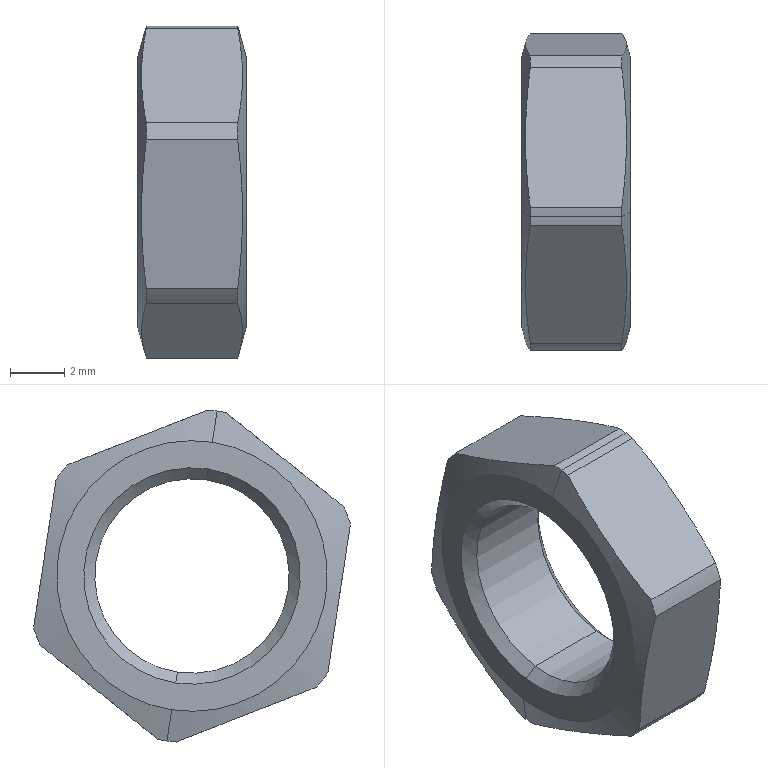Component | SolidWorks | CCDJSACA0806-1-2_CCDJSACA-0806-1_NT-3 | 1 solid | 25 faces | box 4 x 11.71 x 12.27 mm | volume 245 mm3 | cylinder 9 | cone 8 | plane 8 | commonest cylinder face diameters 12.325 x7 7.188 x2
STEP:
#1=CARTESIAN_POINT('',(-8.728,15.708,-2.258));
#2=VERTEX_POINT('',#1);
#3=CARTESIAN_POINT('',(-8.728,15.694,-2.26));
#4=VERTEX_POINT('',#3);
#5=CARTESIAN_POINT('',(-8.728,15.731,-2.5));
#6=DIRECTION('',(1.,-0.,-0.));
#7=DIRECTION('',(0.,-0.1502,0.9887));
#8=AXIS2_PLACEMENT_3D('',#5,#6,#7);
#9=CIRCLE('',#8,0.2426);
#10=EDGE_CURVE('',#2,#4,#9,.T.);
#11=ORIENTED_EDGE('',*,*,#10,.T.);
#12=CARTESIAN_POINT('',(-8.595,15.694,-2.26));
#13=VERTEX_POINT('',#12);
#14=CARTESIAN_POINT('',(-8.898,15.694,-2.26));
#15=DIRECTION('',(1.,-0.,-0.));
#16=VECTOR('',#15,39.37);
#17=LINE('',#14,#16);
#18=EDGE_CURVE('',#4,#13,#17,.T.);
#19=ORIENTED_EDGE('',*,*,#18,.T.);
#20=CARTESIAN_POINT('',(-8.595,15.708,-2.258));
#21=VERTEX_POINT('',#20);
#22=CARTESIAN_POINT('',(-8.595,15.731,-2.5));
#23=DIRECTION('',(-1.,0.,0.));
#24=DIRECTION('',(0.,0.1502,-0.9887));
#25=AXIS2_PLACEMENT_3D('',#22,#23,#24);
#26=CIRCLE('',#25,0.2426);
#27=EDGE_CURVE('',#13,#21,#26,.T.);
#28=ORIENTED_EDGE('',*,*,#27,.T.);
#29=CARTESIAN_POINT('',(-8.898,15.708,-2.258));
#30=DIRECTION('',(1.,-0.,-0.));
#31=VECTOR('',#30,39.37);
#32=LINE('',#29,#31);
#33=EDGE_CURVE('',#2,#21,#32,.T.);
#34=ORIENTED_EDGE('',*,*,#33,.F.);
#35=EDGE_LOOP('',(#11,#19,#28,#34));
#36=FACE_OUTER_BOUND('',#35,.T.);
#37=CARTESIAN_POINT('',(-8.898,15.731,-2.5));
#38=DIRECTION('',(1.,-0.,-0.));
#39=DIRECTION('',(0.,-0.1502,0.9887));
#40=AXIS2_PLACEMENT_3D('',#37,#38,#39);
#41=CYLINDRICAL_SURFACE('',#40,0.2426);
#42=ADVANCED_FACE('',(#36),#41,.T.);
#43=CARTESIAN_POINT('',(-8.724,15.752,-2.64));
#44=VERTEX_POINT('',#43);
#45=CARTESIAN_POINT('',(-8.724,15.71,-2.36));
#46=VERTEX_POINT('',#45);
#47=CARTESIAN_POINT('',(-8.724,15.731,-2.5));
#48=DIRECTION('',(1.,-0.,-0.));
#49=DIRECTION('',(0.,-0.1502,0.9887));
#50=AXIS2_PLACEMENT_3D('',#47,#48,#49);
#51=CIRCLE('',#50,0.1415);
#52=EDGE_CURVE('',#44,#46,#51,.T.);
#53=ORIENTED_EDGE('',*,*,#52,.T.);
#54=CARTESIAN_POINT('',(-8.74,15.707,-2.344));
#55=VERTEX_POINT('',#54);
#56=CARTESIAN_POINT('',(-8.724,15.71,-2.36));
#57=DIRECTION('',(-0.7071,-0.1062,0.6991));
#58=VECTOR('',#57,39.37);
#59=LINE('',#56,#58);
#60=EDGE_CURVE('',#46,#55,#59,.T.);
#61=ORIENTED_EDGE('',*,*,#60,.T.);
#62=CARTESIAN_POINT('',(-8.74,15.755,-2.656));
#63=VERTEX_POINT('',#62);
#64=CARTESIAN_POINT('',(-8.74,15.731,-2.5));
#65=DIRECTION('',(1.,-0.,-0.));
#66=DIRECTION('',(0.,-0.1502,0.9887));
#67=AXIS2_PLACEMENT_3D('',#64,#65,#66);
#68=CIRCLE('',#67,0.1575);
#69=EDGE_CURVE('',#63,#55,#68,.T.);
#70=ORIENTED_EDGE('',*,*,#69,.F.);
#71=CARTESIAN_POINT('',(-8.724,15.752,-2.64));
#72=DIRECTION('',(-0.7071,0.1062,-0.6991));
#73=VECTOR('',#72,39.37);
#74=LINE('',#71,#73);
#75=EDGE_CURVE('',#44,#63,#74,.T.);
#76=ORIENTED_EDGE('',*,*,#75,.F.);
#77=EDGE_LOOP('',(#53,#61,#70,#76));
#78=FACE_OUTER_BOUND('',#77,.T.);
#79=CARTESIAN_POINT('',(-8.724,15.731,-2.5));
#80=DIRECTION('',(-1.,0.,0.));
#81=DIRECTION('',(0.,0.1502,-0.9887));
#82=AXIS2_PLACEMENT_3D('',#79,#80,#81);
#83=CONICAL_SURFACE('',#82,0.1415,0.7854);
#84=ADVANCED_FACE('',(#78),#83,.F.);
#85=ORIENTED_EDGE('',*,*,#52,.F.);
#86=CARTESIAN_POINT('',(-8.599,15.752,-2.64));
#87=VERTEX_POINT('',#86);
#88=CARTESIAN_POINT('',(-8.74,15.752,-2.64));
#89=DIRECTION('',(1.,-0.,-0.));
#90=VECTOR('',#89,39.37);
#91=LINE('',#88,#90);
#92=EDGE_CURVE('',#44,#87,#91,.T.);
#93=ORIENTED_EDGE('',*,*,#92,.T.);
#94=CARTESIAN_POINT('',(-8.599,15.71,-2.36));
#95=VERTEX_POINT('',#94);
#96=CARTESIAN_POINT('',(-8.599,15.731,-2.5));
#97=DIRECTION('',(1.,-0.,-0.));
#98=DIRECTION('',(0.,-0.1502,0.9887));
#99=AXIS2_PLACEMENT_3D('',#96,#97,#98);
#100=CIRCLE('',#99,0.1415);
#101=EDGE_CURVE('',#87,#95,#100,.T.);
#102=ORIENTED_EDGE('',*,*,#101,.T.);
#103=CARTESIAN_POINT('',(-8.74,15.71,-2.36));
#104=DIRECTION('',(1.,-0.,-0.));
#105=VECTOR('',#104,39.37);
#106=LINE('',#103,#105);
#107=EDGE_CURVE('',#46,#95,#106,.T.);
#108=ORIENTED_EDGE('',*,*,#107,.F.);
#109=EDGE_LOOP('',(#85,#93,#102,#108));
#110=FACE_OUTER_BOUND('',#109,.T.);
#111=CARTESIAN_POINT('',(-8.74,15.731,-2.5));
#112=DIRECTION('',(1.,-0.,-0.));
#113=DIRECTION('',(0.,-0.1502,0.9887));
#114=AXIS2_PLACEMENT_3D('',#111,#112,#113);
#115=CYLINDRICAL_SURFACE('',#114,0.1415);
#116=ADVANCED_FACE('',(#110),#115,.F.);
#117=ORIENTED_EDGE('',*,*,#101,.F.);
#118=CARTESIAN_POINT('',(-8.583,15.755,-2.656));
#119=VERTEX_POINT('',#118);
#120=CARTESIAN_POINT('',(-8.583,15.755,-2.656));
#121=DIRECTION('',(0.7071,0.1062,-0.6991));
#122=VECTOR('',#121,39.37);
#123=LINE('',#120,#122);
#124=EDGE_CURVE('',#87,#119,#123,.T.);
#125=ORIENTED_EDGE('',*,*,#124,.T.);
#126=CARTESIAN_POINT('',(-8.583,15.707,-2.344));
#127=VERTEX_POINT('',#126);
#128=CARTESIAN_POINT('',(-8.583,15.731,-2.5));
#129=DIRECTION('',(1.,-0.,-0.));
#130=DIRECTION('',(0.,-0.1502,0.9887));
#131=AXIS2_PLACEMENT_3D('',#128,#129,#130);
#132=CIRCLE('',#131,0.1575);
#133=EDGE_CURVE('',#119,#127,#132,.T.);
#134=ORIENTED_EDGE('',*,*,#133,.T.);
#135=CARTESIAN_POINT('',(-8.583,15.707,-2.344));
#136=DIRECTION('',(0.7071,-0.1062,0.6991));
#137=VECTOR('',#136,39.37);
#138=LINE('',#135,#137);
#139=EDGE_CURVE('',#95,#127,#138,.T.);
#140=ORIENTED_EDGE('',*,*,#139,.F.);
#141=EDGE_LOOP('',(#117,#125,#134,#140));
#142=FACE_OUTER_BOUND('',#141,.T.);
#143=CARTESIAN_POINT('',(-8.583,15.731,-2.5));
#144=DIRECTION('',(1.,-0.,-0.));
#145=DIRECTION('',(0.,-0.1502,0.9887));
#146=AXIS2_PLACEMENT_3D('',#143,#144,#145);
#147=CONICAL_SURFACE('',#146,0.1575,0.7854);
#148=ADVANCED_FACE('',(#142),#147,.F.);
#149=CARTESIAN_POINT('',(-8.583,15.701,-2.305));
#150=VERTEX_POINT('',#149);
#151=CARTESIAN_POINT('',(-8.583,15.76,-2.695));
#152=VERTEX_POINT('',#151);
#153=CARTESIAN_POINT('',(-8.583,15.731,-2.5));
#154=DIRECTION('',(1.,-0.,-0.));
#155=DIRECTION('',(0.,-0.1502,0.9887));
#156=AXIS2_PLACEMENT_3D('',#153,#154,#155);
#157=CIRCLE('',#156,0.1969);
#158=EDGE_CURVE('',#150,#152,#157,.T.);
#159=ORIENTED_EDGE('',*,*,#158,.F.);
#160=CARTESIAN_POINT('',(-8.661,15.657,-2.015));
#161=DIRECTION('',(-0.2588,-0.1451,0.955));
#162=VECTOR('',#161,39.37);
#163=LINE('',#160,#162);
#164=EDGE_CURVE('',#150,#13,#163,.T.);
#165=ORIENTED_EDGE('',*,*,#164,.T.);
#166=CARTESIAN_POINT('',(-8.595,15.681,-2.263));
#167=VERTEX_POINT('',#166);
#168=CARTESIAN_POINT('',(-8.595,15.731,-2.5));
#169=DIRECTION('',(-1.,0.,0.));
#170=DIRECTION('',(0.,0.1502,-0.9887));
#171=AXIS2_PLACEMENT_3D('',#168,#169,#170);
#172=CIRCLE('',#171,0.2426);
#173=EDGE_CURVE('',#167,#13,#172,.T.);
#174=ORIENTED_EDGE('',*,*,#173,.F.);
#175=CARTESIAN_POINT('',(-8.595,15.51,-2.399));
#176=VERTEX_POINT('',#175);
#177=CARTESIAN_POINT('',(-8.595,15.51,-2.399));
#178=CARTESIAN_POINT('',(-8.591,15.539,-2.376));
#179=CARTESIAN_POINT('',(-8.585,15.596,-2.331));
#180=CARTESIAN_POINT('',(-8.591,15.653,-2.285));
#181=CARTESIAN_POINT('',(-8.595,15.681,-2.263));
#182=B_SPLINE_CURVE_WITH_KNOTS('',3,(#177,#178,#179,#180,#181),.UNSPECIFIED.,.F.,.F.,(4,1,4),(0.0003961,0.003176,0.005955),.UNSPECIFIED.);
#183=EDGE_CURVE('',#176,#167,#182,.T.);
#184=ORIENTED_EDGE('',*,*,#183,.F.);
#185=CARTESIAN_POINT('',(-8.595,15.5,-2.424));
#186=VERTEX_POINT('',#185);
#187=CARTESIAN_POINT('',(-8.595,15.731,-2.5));
#188=DIRECTION('',(-1.,0.,0.));
#189=DIRECTION('',(0.,0.1502,-0.9887));
#190=AXIS2_PLACEMENT_3D('',#187,#188,#189);
#191=CIRCLE('',#190,0.2426);
#192=EDGE_CURVE('',#186,#176,#191,.T.);
#193=ORIENTED_EDGE('',*,*,#192,.F.);
#194=CARTESIAN_POINT('',(-8.595,15.533,-2.641));
#195=VERTEX_POINT('',#194);
#196=CARTESIAN_POINT('',(-8.595,15.533,-2.641));
#197=CARTESIAN_POINT('',(-8.591,15.528,-2.605));
#198=CARTESIAN_POINT('',(-8.588,15.522,-2.568));
#199=CARTESIAN_POINT('',(-8.588,15.511,-2.496));
#200=CARTESIAN_POINT('',(-8.591,15.506,-2.46));
#201=CARTESIAN_POINT('',(-8.595,15.5,-2.424));
#202=B_SPLINE_CURVE_WITH_KNOTS('',3,(#196,#197,#198,#199,#200,#201),.UNSPECIFIED.,.F.,.F.,(4,2,4),(0.005822,0.00862,0.01142),.UNSPECIFIED.);
#203=EDGE_CURVE('',#195,#186,#202,.T.);
#204=ORIENTED_EDGE('',*,*,#203,.F.);
#205=CARTESIAN_POINT('',(-8.595,15.55,-2.662));
#206=VERTEX_POINT('',#205);
#207=CARTESIAN_POINT('',(-8.595,15.731,-2.5));
#208=DIRECTION('',(-1.,0.,0.));
#209=DIRECTION('',(0.,0.1502,-0.9887));
#210=AXIS2_PLACEMENT_3D('',#207,#208,#209);
#211=CIRCLE('',#210,0.2426);
#212=EDGE_CURVE('',#206,#195,#211,.T.);
#213=ORIENTED_EDGE('',*,*,#212,.F.);
#214=CARTESIAN_POINT('',(-8.595,15.754,-2.742));
#215=VERTEX_POINT('',#214);
#216=CARTESIAN_POINT('',(-8.595,15.754,-2.742));
#217=CARTESIAN_POINT('',(-8.591,15.72,-2.728));
#218=CARTESIAN_POINT('',(-8.585,15.652,-2.702));
#219=CARTESIAN_POINT('',(-8.591,15.584,-2.675));
#220=CARTESIAN_POINT('',(-8.595,15.55,-2.662));
#221=B_SPLINE_CURVE_WITH_KNOTS('',3,(#216,#217,#218,#219,#220),.UNSPECIFIED.,.F.,.F.,(4,1,4),(0.0003961,0.003176,0.005955),.UNSPECIFIED.);
#222=EDGE_CURVE('',#215,#206,#221,.T.);
#223=ORIENTED_EDGE('',*,*,#222,.F.);
#224=CARTESIAN_POINT('',(-8.595,15.767,-2.74));
#225=VERTEX_POINT('',#224);
#226=CARTESIAN_POINT('',(-8.595,15.731,-2.5));
#227=DIRECTION('',(-1.,0.,0.));
#228=DIRECTION('',(0.,0.1502,-0.9887));
#229=AXIS2_PLACEMENT_3D('',#226,#227,#228);
#230=CIRCLE('',#229,0.2426);
#231=EDGE_CURVE('',#225,#215,#230,.T.);
#232=ORIENTED_EDGE('',*,*,#231,.F.);
#233=CARTESIAN_POINT('',(-8.661,15.805,-2.985));
#234=DIRECTION('',(-0.2588,0.1451,-0.955));
#235=VECTOR('',#234,39.37);
#236=LINE('',#233,#235);
#237=EDGE_CURVE('',#152,#225,#236,.T.);
#238=ORIENTED_EDGE('',*,*,#237,.F.);
#239=EDGE_LOOP('',(#159,#165,#174,#184,#193,#204,#213,#223,#232,#238));
#240=FACE_OUTER_BOUND('',#239,.T.);
#241=CARTESIAN_POINT('',(-8.661,15.731,-2.5));
#242=DIRECTION('',(-1.,0.,0.));
#243=DIRECTION('',(0.,0.1502,-0.9887));
#244=AXIS2_PLACEMENT_3D('',#241,#242,#243);
#245=CONICAL_SURFACE('',#244,0.4907,1.309);
#246=ADVANCED_FACE('',(#240),#245,.T.);
#247=CARTESIAN_POINT('',(-8.74,15.701,-2.305));
#248=VERTEX_POINT('',#247);
#249=CARTESIAN_POINT('',(-8.74,15.76,-2.695));
#250=VERTEX_POINT('',#249);
#251=CARTESIAN_POINT('',(-8.74,15.731,-2.5));
#252=DIRECTION('',(1.,-0.,-0.));
#253=DIRECTION('',(0.,-0.1502,0.9887));
#254=AXIS2_PLACEMENT_3D('',#251,#252,#253);
#255=CIRCLE('',#254,0.1969);
#256=EDGE_CURVE('',#248,#250,#255,.T.);
#257=ORIENTED_EDGE('',*,*,#256,.T.);
#258=CARTESIAN_POINT('',(-8.728,15.767,-2.74));
#259=VERTEX_POINT('',#258);
#260=CARTESIAN_POINT('',(-8.74,15.76,-2.695));
#261=DIRECTION('',(0.2588,0.1451,-0.955));
#262=VECTOR('',#261,39.37);
#263=LINE('',#260,#262);
#264=EDGE_CURVE('',#250,#259,#263,.T.);
#265=ORIENTED_EDGE('',*,*,#264,.T.);
#266=CARTESIAN_POINT('',(-8.728,15.754,-2.742));
#267=VERTEX_POINT('',#266);
#268=CARTESIAN_POINT('',(-8.728,15.731,-2.5));
#269=DIRECTION('',(1.,-0.,-0.));
#270=DIRECTION('',(0.,-0.1502,0.9887));
#271=AXIS2_PLACEMENT_3D('',#268,#269,#270);
#272=CIRCLE('',#271,0.2426);
#273=EDGE_CURVE('',#267,#259,#272,.T.);
#274=ORIENTED_EDGE('',*,*,#273,.F.);
#275=CARTESIAN_POINT('',(-8.728,15.55,-2.662));
#276=VERTEX_POINT('',#275);
#277=CARTESIAN_POINT('',(-8.728,15.55,-2.662));
#278=CARTESIAN_POINT('',(-8.732,15.584,-2.675));
#279=CARTESIAN_POINT('',(-8.737,15.652,-2.702));
#280=CARTESIAN_POINT('',(-8.732,15.72,-2.728));
#281=CARTESIAN_POINT('',(-8.728,15.754,-2.742));
#282=B_SPLINE_CURVE_WITH_KNOTS('',3,(#277,#278,#279,#280,#281),.UNSPECIFIED.,.F.,.F.,(4,1,4),(0.0003961,0.003176,0.005955),.UNSPECIFIED.);
#283=EDGE_CURVE('',#276,#267,#282,.T.);
#284=ORIENTED_EDGE('',*,*,#283,.F.);
#285=CARTESIAN_POINT('',(-8.728,15.533,-2.641));
#286=VERTEX_POINT('',#285);
#287=CARTESIAN_POINT('',(-8.728,15.731,-2.5));
#288=DIRECTION('',(1.,-0.,-0.));
#289=DIRECTION('',(0.,-0.1502,0.9887));
#290=AXIS2_PLACEMENT_3D('',#287,#288,#289);
#291=CIRCLE('',#290,0.2426);
#292=EDGE_CURVE('',#286,#276,#291,.T.);
#293=ORIENTED_EDGE('',*,*,#292,.F.);
#294=CARTESIAN_POINT('',(-8.728,15.5,-2.424));
#295=VERTEX_POINT('',#294);
#296=CARTESIAN_POINT('',(-8.728,15.5,-2.424));
#297=CARTESIAN_POINT('',(-8.732,15.506,-2.46));
#298=CARTESIAN_POINT('',(-8.735,15.511,-2.496));
#299=CARTESIAN_POINT('',(-8.735,15.522,-2.568));
#300=CARTESIAN_POINT('',(-8.732,15.528,-2.605));
#301=CARTESIAN_POINT('',(-8.728,15.533,-2.641));
#302=B_SPLINE_CURVE_WITH_KNOTS('',3,(#296,#297,#298,#299,#300,#301),.UNSPECIFIED.,.F.,.F.,(4,2,4),(0.0139,0.01669,0.01948),.UNSPECIFIED.);
#303=EDGE_CURVE('',#295,#286,#302,.T.);
#304=ORIENTED_EDGE('',*,*,#303,.F.);
#305=CARTESIAN_POINT('',(-8.728,15.51,-2.399));
#306=VERTEX_POINT('',#305);
#307=CARTESIAN_POINT('',(-8.728,15.731,-2.5));
#308=DIRECTION('',(1.,-0.,-0.));
#309=DIRECTION('',(0.,-0.1502,0.9887));
#310=AXIS2_PLACEMENT_3D('',#307,#308,#309);
#311=CIRCLE('',#310,0.2426);
#312=EDGE_CURVE('',#306,#295,#311,.T.);
#313=ORIENTED_EDGE('',*,*,#312,.F.);
#314=CARTESIAN_POINT('',(-8.728,15.681,-2.263));
#315=VERTEX_POINT('',#314);
#316=CARTESIAN_POINT('',(-8.728,15.681,-2.263));
#317=CARTESIAN_POINT('',(-8.732,15.653,-2.285));
#318=CARTESIAN_POINT('',(-8.737,15.596,-2.331));
#319=CARTESIAN_POINT('',(-8.732,15.539,-2.376));
#320=CARTESIAN_POINT('',(-8.728,15.51,-2.399));
#321=B_SPLINE_CURVE_WITH_KNOTS('',3,(#316,#317,#318,#319,#320),.UNSPECIFIED.,.F.,.F.,(4,1,4),(0.0003961,0.003176,0.005955),.UNSPECIFIED.);
#322=EDGE_CURVE('',#315,#306,#321,.T.);
#323=ORIENTED_EDGE('',*,*,#322,.F.);
#324=CARTESIAN_POINT('',(-8.728,15.731,-2.5));
#325=DIRECTION('',(1.,-0.,-0.));
#326=DIRECTION('',(0.,-0.1502,0.9887));
#327=AXIS2_PLACEMENT_3D('',#324,#325,#326);
#328=CIRCLE('',#327,0.2426);
#329=EDGE_CURVE('',#4,#315,#328,.T.);
#330=ORIENTED_EDGE('',*,*,#329,.F.);
#331=CARTESIAN_POINT('',(-8.74,15.701,-2.305));
#332=DIRECTION('',(0.2588,-0.1451,0.955));
#333=VECTOR('',#332,39.37);
#334=LINE('',#331,#333);
#335=EDGE_CURVE('',#248,#4,#334,.T.);
#336=ORIENTED_EDGE('',*,*,#335,.F.);
#337=EDGE_LOOP('',(#257,#265,#274,#284,#293,#304,#313,#323,#330,#336));
#338=FACE_OUTER_BOUND('',#337,.T.);
#339=CARTESIAN_POINT('',(-8.74,15.731,-2.5));
#340=DIRECTION('',(1.,-0.,-0.));
#341=DIRECTION('',(0.,-0.1502,0.9887));
#342=AXIS2_PLACEMENT_3D('',#339,#340,#341);
#343=CONICAL_SURFACE('',#342,0.1969,1.309);
#344=ADVANCED_FACE('',(#338),#343,.T.);
#345=ORIENTED_EDGE('',*,*,#264,.F.);
#346=CARTESIAN_POINT('',(-8.74,15.731,-2.5));
#347=DIRECTION('',(1.,-0.,-0.));
#348=DIRECTION('',(0.,-0.1502,0.9887));
#349=AXIS2_PLACEMENT_3D('',#346,#347,#348);
#350=CIRCLE('',#349,0.1969);
#351=EDGE_CURVE('',#250,#248,#350,.T.);
#352=ORIENTED_EDGE('',*,*,#351,.T.);
#353=ORIENTED_EDGE('',*,*,#335,.T.);
#354=ORIENTED_EDGE('',*,*,#10,.F.);
#355=CARTESIAN_POINT('',(-8.728,15.912,-2.338));
#356=VERTEX_POINT('',#355);
#357=CARTESIAN_POINT('',(-8.728,15.912,-2.338));
#358=CARTESIAN_POINT('',(-8.732,15.878,-2.325));
#359=CARTESIAN_POINT('',(-8.737,15.81,-2.298));
#360=CARTESIAN_POINT('',(-8.732,15.742,-2.272));
#361=CARTESIAN_POINT('',(-8.728,15.708,-2.258));
#362=B_SPLINE_CURVE_WITH_KNOTS('',3,(#357,#358,#359,#360,#361),.UNSPECIFIED.,.F.,.F.,(4,1,4),(0.0003961,0.003176,0.005955),.UNSPECIFIED.);
#363=EDGE_CURVE('',#356,#2,#362,.T.);
#364=ORIENTED_EDGE('',*,*,#363,.F.);
#365=CARTESIAN_POINT('',(-8.728,15.929,-2.359));
#366=VERTEX_POINT('',#365);
#367=CARTESIAN_POINT('',(-8.728,15.731,-2.5));
#368=DIRECTION('',(1.,-0.,-0.));
#369=DIRECTION('',(0.,-0.1502,0.9887));
#370=AXIS2_PLACEMENT_3D('',#367,#368,#369);
#371=CIRCLE('',#370,0.2426);
#372=EDGE_CURVE('',#366,#356,#371,.T.);
#373=ORIENTED_EDGE('',*,*,#372,.F.);
#374=CARTESIAN_POINT('',(-8.728,15.961,-2.576));
#375=VERTEX_POINT('',#374);
#376=CARTESIAN_POINT('',(-8.728,15.961,-2.576));
#377=CARTESIAN_POINT('',(-8.732,15.956,-2.54));
#378=CARTESIAN_POINT('',(-8.735,15.95,-2.503));
#379=CARTESIAN_POINT('',(-8.735,15.939,-2.431));
#380=CARTESIAN_POINT('',(-8.732,15.934,-2.395));
#381=CARTESIAN_POINT('',(-8.728,15.929,-2.359));
#382=B_SPLINE_CURVE_WITH_KNOTS('',3,(#376,#377,#378,#379,#380,#381),.UNSPECIFIED.,.F.,.F.,(4,2,4),(0.005822,0.00862,0.01142),.UNSPECIFIED.);
#383=EDGE_CURVE('',#375,#366,#382,.T.);
#384=ORIENTED_EDGE('',*,*,#383,.F.);
#385=CARTESIAN_POINT('',(-8.728,15.952,-2.601));
#386=VERTEX_POINT('',#385);
#387=CARTESIAN_POINT('',(-8.728,15.731,-2.5));
#388=DIRECTION('',(1.,-0.,-0.));
#389=DIRECTION('',(0.,-0.1502,0.9887));
#390=AXIS2_PLACEMENT_3D('',#387,#388,#389);
#391=CIRCLE('',#390,0.2426);
#392=EDGE_CURVE('',#386,#375,#391,.T.);
#393=ORIENTED_EDGE('',*,*,#392,.F.);
#394=CARTESIAN_POINT('',(-8.728,15.781,-2.737));
#395=VERTEX_POINT('',#394);
#396=CARTESIAN_POINT('',(-8.728,15.781,-2.737));
#397=CARTESIAN_POINT('',(-8.732,15.809,-2.715));
#398=CARTESIAN_POINT('',(-8.737,15.866,-2.669));
#399=CARTESIAN_POINT('',(-8.732,15.923,-2.624));
#400=CARTESIAN_POINT('',(-8.728,15.952,-2.601));
#401=B_SPLINE_CURVE_WITH_KNOTS('',3,(#396,#397,#398,#399,#400),.UNSPECIFIED.,.F.,.F.,(4,1,4),(0.0003961,0.003176,0.005955),.UNSPECIFIED.);
#402=EDGE_CURVE('',#395,#386,#401,.T.);
#403=ORIENTED_EDGE('',*,*,#402,.F.);
#404=CARTESIAN_POINT('',(-8.728,15.731,-2.5));
#405=DIRECTION('',(1.,-0.,-0.));
#406=DIRECTION('',(0.,-0.1502,0.9887));
#407=AXIS2_PLACEMENT_3D('',#404,#405,#406);
#408=CIRCLE('',#407,0.2426);
#409=EDGE_CURVE('',#259,#395,#408,.T.);
#410=ORIENTED_EDGE('',*,*,#409,.F.);
#411=EDGE_LOOP('',(#345,#352,#353,#354,#364,#373,#384,#393,#403,#410));
#412=FACE_OUTER_BOUND('',#411,.T.);
#413=CARTESIAN_POINT('',(-8.74,15.731,-2.5));
#414=DIRECTION('',(1.,-0.,-0.));
#415=DIRECTION('',(0.,-0.1502,0.9887));
#416=AXIS2_PLACEMENT_3D('',#413,#414,#415);
#417=CONICAL_SURFACE('',#416,0.1969,1.309);
#418=ADVANCED_FACE('',(#412),#417,.T.);
#419=ORIENTED_EDGE('',*,*,#164,.F.);
#420=CARTESIAN_POINT('',(-8.583,15.731,-2.5));
#421=DIRECTION('',(1.,-0.,-0.));
#422=DIRECTION('',(0.,-0.1502,0.9887));
#423=AXIS2_PLACEMENT_3D('',#420,#421,#422);
#424=CIRCLE('',#423,0.1969);
#425=EDGE_CURVE('',#152,#150,#424,.T.);
#426=ORIENTED_EDGE('',*,*,#425,.F.);
#427=ORIENTED_EDGE('',*,*,#237,.T.);
#428=CARTESIAN_POINT('',(-8.595,15.781,-2.737));
#429=VERTEX_POINT('',#428);
#430=CARTESIAN_POINT('',(-8.595,15.731,-2.5));
#431=DIRECTION('',(-1.,0.,0.));
#432=DIRECTION('',(0.,0.1502,-0.9887));
#433=AXIS2_PLACEMENT_3D('',#430,#431,#432);
#434=CIRCLE('',#433,0.2426);
#435=EDGE_CURVE('',#429,#225,#434,.T.);
#436=ORIENTED_EDGE('',*,*,#435,.F.);
#437=CARTESIAN_POINT('',(-8.595,15.952,-2.601));
#438=VERTEX_POINT('',#437);
#439=CARTESIAN_POINT('',(-8.595,15.952,-2.601));
#440=CARTESIAN_POINT('',(-8.591,15.923,-2.624));
#441=CARTESIAN_POINT('',(-8.585,15.866,-2.669));
#442=CARTESIAN_POINT('',(-8.591,15.809,-2.715));
#443=CARTESIAN_POINT('',(-8.595,15.781,-2.737));
#444=B_SPLINE_CURVE_WITH_KNOTS('',3,(#439,#440,#441,#442,#443),.UNSPECIFIED.,.F.,.F.,(4,1,4),(0.0003961,0.003176,0.005955),.UNSPECIFIED.);
#445=EDGE_CURVE('',#438,#429,#444,.T.);
#446=ORIENTED_EDGE('',*,*,#445,.F.);
#447=CARTESIAN_POINT('',(-8.595,15.961,-2.576));
#448=VERTEX_POINT('',#447);
#449=CARTESIAN_POINT('',(-8.595,15.731,-2.5));
#450=DIRECTION('',(-1.,0.,0.));
#451=DIRECTION('',(0.,0.1502,-0.9887));
#452=AXIS2_PLACEMENT_3D('',#449,#450,#451);
#453=CIRCLE('',#452,0.2426);
#454=EDGE_CURVE('',#448,#438,#453,.T.);
#455=ORIENTED_EDGE('',*,*,#454,.F.);
#456=CARTESIAN_POINT('',(-8.595,15.929,-2.359));
#457=VERTEX_POINT('',#456);
#458=CARTESIAN_POINT('',(-8.595,15.929,-2.359));
#459=CARTESIAN_POINT('',(-8.591,15.934,-2.395));
#460=CARTESIAN_POINT('',(-8.588,15.939,-2.431));
#461=CARTESIAN_POINT('',(-8.588,15.95,-2.503));
#462=CARTESIAN_POINT('',(-8.591,15.956,-2.54));
#463=CARTESIAN_POINT('',(-8.595,15.961,-2.576));
#464=B_SPLINE_CURVE_WITH_KNOTS('',3,(#458,#459,#460,#461,#462,#463),.UNSPECIFIED.,.F.,.F.,(4,2,4),(0.0139,0.01669,0.01948),.UNSPECIFIED.);
#465=EDGE_CURVE('',#457,#448,#464,.T.);
#466=ORIENTED_EDGE('',*,*,#465,.F.);
#467=CARTESIAN_POINT('',(-8.595,15.912,-2.338));
#468=VERTEX_POINT('',#467);
#469=CARTESIAN_POINT('',(-8.595,15.731,-2.5));
#470=DIRECTION('',(-1.,0.,0.));
#471=DIRECTION('',(0.,0.1502,-0.9887));
#472=AXIS2_PLACEMENT_3D('',#469,#470,#471);
#473=CIRCLE('',#472,0.2426);
#474=EDGE_CURVE('',#468,#457,#473,.T.);
#475=ORIENTED_EDGE('',*,*,#474,.F.);
#476=CARTESIAN_POINT('',(-8.595,15.708,-2.258));
#477=CARTESIAN_POINT('',(-8.591,15.742,-2.272));
#478=CARTESIAN_POINT('',(-8.585,15.81,-2.298));
#479=CARTESIAN_POINT('',(-8.591,15.878,-2.325));
#480=CARTESIAN_POINT('',(-8.595,15.912,-2.338));
#481=B_SPLINE_CURVE_WITH_KNOTS('',3,(#476,#477,#478,#479,#480),.UNSPECIFIED.,.F.,.F.,(4,1,4),(0.0003961,0.003176,0.005955),.UNSPECIFIED.);
#482=EDGE_CURVE('',#21,#468,#481,.T.);
#483=ORIENTED_EDGE('',*,*,#482,.F.);
#484=ORIENTED_EDGE('',*,*,#27,.F.);
#485=EDGE_LOOP('',(#419,#426,#427,#436,#446,#455,#466,#475,#483,#484));
#486=FACE_OUTER_BOUND('',#485,.T.);
#487=CARTESIAN_POINT('',(-8.661,15.731,-2.5));
#488=DIRECTION('',(-1.,0.,0.));
#489=DIRECTION('',(0.,0.1502,-0.9887));
#490=AXIS2_PLACEMENT_3D('',#487,#488,#489);
#491=CONICAL_SURFACE('',#490,0.4907,1.309);
#492=ADVANCED_FACE('',(#486),#491,.T.);
#493=ORIENTED_EDGE('',*,*,#402,.T.);
#494=CARTESIAN_POINT('',(-8.898,15.952,-2.601));
#495=DIRECTION('',(1.,-0.,-0.));
#496=VECTOR('',#495,39.37);
#497=LINE('',#494,#496);
#498=EDGE_CURVE('',#386,#438,#497,.T.);
#499=ORIENTED_EDGE('',*,*,#498,.T.);
#500=ORIENTED_EDGE('',*,*,#445,.T.);
#501=CARTESIAN_POINT('',(-8.898,15.781,-2.737));
#502=DIRECTION('',(-1.,0.,0.));
#503=VECTOR('',#502,39.37);
#504=LINE('',#501,#503);
#505=EDGE_CURVE('',#429,#395,#504,.T.);
#506=ORIENTED_EDGE('',*,*,#505,.T.);
#507=EDGE_LOOP('',(#493,#499,#500,#506));
#508=FACE_OUTER_BOUND('',#507,.T.);
#509=CARTESIAN_POINT('',(-8.898,15.768,-2.747));
#510=DIRECTION('',(0.,0.6244,-0.7811));
#511=DIRECTION('',(0.,0.7811,0.6244));
#512=AXIS2_PLACEMENT_3D('',#509,#510,#511);
#513=PLANE('',#512);
#514=ADVANCED_FACE('',(#508),#513,.T.);
#515=ORIENTED_EDGE('',*,*,#283,.T.);
#516=CARTESIAN_POINT('',(-8.898,15.754,-2.742));
#517=DIRECTION('',(1.,-0.,-0.));
#518=VECTOR('',#517,39.37);
#519=LINE('',#516,#518);
#520=EDGE_CURVE('',#267,#215,#519,.T.);
#521=ORIENTED_EDGE('',*,*,#520,.T.);
#522=ORIENTED_EDGE('',*,*,#222,.T.);
#523=CARTESIAN_POINT('',(-8.898,15.55,-2.662));
#524=DIRECTION('',(-1.,0.,0.));
#525=VECTOR('',#524,39.37);
#526=LINE('',#523,#525);
#527=EDGE_CURVE('',#206,#276,#526,.T.);
#528=ORIENTED_EDGE('',*,*,#527,.T.);
#529=EDGE_LOOP('',(#515,#521,#522,#528));
#530=FACE_OUTER_BOUND('',#529,.T.);
#531=CARTESIAN_POINT('',(-8.898,15.536,-2.656));
#532=DIRECTION('',(-0.,-0.3642,-0.9313));
#533=DIRECTION('',(0.,0.9313,-0.3642));
#534=AXIS2_PLACEMENT_3D('',#531,#532,#533);
#535=PLANE('',#534);
#536=ADVANCED_FACE('',(#530),#535,.T.);
#537=ORIENTED_EDGE('',*,*,#303,.T.);
#538=CARTESIAN_POINT('',(-8.898,15.533,-2.641));
#539=DIRECTION('',(1.,-0.,-0.));
#540=VECTOR('',#539,39.37);
#541=LINE('',#538,#540);
#542=EDGE_CURVE('',#286,#195,#541,.T.);
#543=ORIENTED_EDGE('',*,*,#542,.T.);
#544=ORIENTED_EDGE('',*,*,#203,.T.);
#545=CARTESIAN_POINT('',(-8.898,15.5,-2.424));
#546=DIRECTION('',(-1.,0.,0.));
#547=VECTOR('',#546,39.37);
#548=LINE('',#545,#547);
#549=EDGE_CURVE('',#186,#295,#548,.T.);
#550=ORIENTED_EDGE('',*,*,#549,.T.);
#551=EDGE_LOOP('',(#537,#543,#544,#550));
#552=FACE_OUTER_BOUND('',#551,.T.);
#553=CARTESIAN_POINT('',(-8.898,15.498,-2.409));
#554=DIRECTION('',(-0.,-0.9887,-0.1502));
#555=DIRECTION('',(0.,0.1502,-0.9887));
#556=AXIS2_PLACEMENT_3D('',#553,#554,#555);
#557=PLANE('',#556);
#558=ADVANCED_FACE('',(#552),#557,.T.);
#559=ORIENTED_EDGE('',*,*,#322,.T.);
#560=CARTESIAN_POINT('',(-8.898,15.51,-2.399));
#561=DIRECTION('',(1.,-0.,-0.));
#562=VECTOR('',#561,39.37);
#563=LINE('',#560,#562);
#564=EDGE_CURVE('',#306,#176,#563,.T.);
#565=ORIENTED_EDGE('',*,*,#564,.T.);
#566=ORIENTED_EDGE('',*,*,#183,.T.);
#567=CARTESIAN_POINT('',(-8.898,15.681,-2.263));
#568=DIRECTION('',(-1.,0.,0.));
#569=VECTOR('',#568,39.37);
#570=LINE('',#567,#569);
#571=EDGE_CURVE('',#167,#315,#570,.T.);
#572=ORIENTED_EDGE('',*,*,#571,.T.);
#573=EDGE_LOOP('',(#559,#565,#566,#572));
#574=FACE_OUTER_BOUND('',#573,.T.);
#575=CARTESIAN_POINT('',(-8.898,15.693,-2.253));
#576=DIRECTION('',(-0.,-0.6244,0.7811));
#577=DIRECTION('',(-0.,-0.7811,-0.6244));
#578=AXIS2_PLACEMENT_3D('',#575,#576,#577);
#579=PLANE('',#578);
#580=ADVANCED_FACE('',(#574),#579,.T.);
#581=ORIENTED_EDGE('',*,*,#363,.T.);
#582=ORIENTED_EDGE('',*,*,#33,.T.);
#583=ORIENTED_EDGE('',*,*,#482,.T.);
#584=CARTESIAN_POINT('',(-8.898,15.912,-2.338));
#585=DIRECTION('',(-1.,0.,0.));
#586=VECTOR('',#585,39.37);
#587=LINE('',#584,#586);
#588=EDGE_CURVE('',#468,#356,#587,.T.);
#589=ORIENTED_EDGE('',*,*,#588,.T.);
#590=EDGE_LOOP('',(#581,#582,#583,#589));
#591=FACE_OUTER_BOUND('',#590,.T.);
#592=CARTESIAN_POINT('',(-8.898,15.926,-2.344));
#593=DIRECTION('',(0.,0.3642,0.9313));
#594=DIRECTION('',(-0.,-0.9313,0.3642));
#595=AXIS2_PLACEMENT_3D('',#592,#593,#594);
#596=PLANE('',#595);
#597=ADVANCED_FACE('',(#591),#596,.T.);
#598=ORIENTED_EDGE('',*,*,#383,.T.);
#599=CARTESIAN_POINT('',(-8.898,15.929,-2.359));
#600=DIRECTION('',(1.,-0.,-0.));
#601=VECTOR('',#600,39.37);
#602=LINE('',#599,#601);
#603=EDGE_CURVE('',#366,#457,#602,.T.);
#604=ORIENTED_EDGE('',*,*,#603,.T.);
#605=ORIENTED_EDGE('',*,*,#465,.T.);
#606=CARTESIAN_POINT('',(-8.898,15.961,-2.576));
#607=DIRECTION('',(-1.,0.,0.));
#608=VECTOR('',#607,39.37);
#609=LINE('',#606,#608);
#610=EDGE_CURVE('',#448,#375,#609,.T.);
#611=ORIENTED_EDGE('',*,*,#610,.T.);
#612=EDGE_LOOP('',(#598,#604,#605,#611));
#613=FACE_OUTER_BOUND('',#612,.T.);
#614=CARTESIAN_POINT('',(-8.898,15.964,-2.591));
#615=DIRECTION('',(0.,0.9887,0.1502));
#616=DIRECTION('',(-0.,-0.1502,0.9887));
#617=AXIS2_PLACEMENT_3D('',#614,#615,#616);
#618=PLANE('',#617);
#619=ADVANCED_FACE('',(#613),#618,.T.);
#620=ORIENTED_EDGE('',*,*,#124,.F.);
#621=CARTESIAN_POINT('',(-8.599,15.731,-2.5));
#622=DIRECTION('',(1.,-0.,-0.));
#623=DIRECTION('',(0.,-0.1502,0.9887));
#624=AXIS2_PLACEMENT_3D('',#621,#622,#623);
#625=CIRCLE('',#624,0.1415);
#626=EDGE_CURVE('',#95,#87,#625,.T.);
#627=ORIENTED_EDGE('',*,*,#626,.F.);
#628=ORIENTED_EDGE('',*,*,#139,.T.);
#629=CARTESIAN_POINT('',(-8.583,15.731,-2.5));
#630=DIRECTION('',(1.,-0.,-0.));
#631=DIRECTION('',(0.,-0.1502,0.9887));
#632=AXIS2_PLACEMENT_3D('',#629,#630,#631);
#633=CIRCLE('',#632,0.1575);
#634=EDGE_CURVE('',#127,#119,#633,.T.);
#635=ORIENTED_EDGE('',*,*,#634,.T.);
#636=EDGE_LOOP('',(#620,#627,#628,#635));
#637=FACE_OUTER_BOUND('',#636,.T.);
#638=CARTESIAN_POINT('',(-8.583,15.731,-2.5));
#639=DIRECTION('',(1.,-0.,-0.));
#640=DIRECTION('',(0.,-0.1502,0.9887));
#641=AXIS2_PLACEMENT_3D('',#638,#639,#640);
#642=CONICAL_SURFACE('',#641,0.1575,0.7854);
#643=ADVANCED_FACE('',(#637),#642,.F.);
#644=ORIENTED_EDGE('',*,*,#92,.F.);
#645=CARTESIAN_POINT('',(-8.724,15.731,-2.5));
#646=DIRECTION('',(1.,-0.,-0.));
#647=DIRECTION('',(0.,-0.1502,0.9887));
#648=AXIS2_PLACEMENT_3D('',#645,#646,#647);
#649=CIRCLE('',#648,0.1415);
#650=EDGE_CURVE('',#46,#44,#649,.T.);
#651=ORIENTED_EDGE('',*,*,#650,.F.);
#652=ORIENTED_EDGE('',*,*,#107,.T.);
#653=ORIENTED_EDGE('',*,*,#626,.T.);
#654=EDGE_LOOP('',(#644,#651,#652,#653));
#655=FACE_OUTER_BOUND('',#654,.T.);
#656=CARTESIAN_POINT('',(-8.74,15.731,-2.5));
#657=DIRECTION('',(1.,-0.,-0.));
#658=DIRECTION('',(0.,-0.1502,0.9887));
#659=AXIS2_PLACEMENT_3D('',#656,#657,#658);
#660=CYLINDRICAL_SURFACE('',#659,0.1415);
#661=ADVANCED_FACE('',(#655),#660,.F.);
#662=ORIENTED_EDGE('',*,*,#60,.F.);
#663=ORIENTED_EDGE('',*,*,#650,.T.);
#664=ORIENTED_EDGE('',*,*,#75,.T.);
#665=CARTESIAN_POINT('',(-8.74,15.731,-2.5));
#666=DIRECTION('',(1.,-0.,-0.));
#667=DIRECTION('',(0.,-0.1502,0.9887));
#668=AXIS2_PLACEMENT_3D('',#665,#666,#667);
#669=CIRCLE('',#668,0.1575);
#670=EDGE_CURVE('',#55,#63,#669,.T.);
#671=ORIENTED_EDGE('',*,*,#670,.F.);
#672=EDGE_LOOP('',(#662,#663,#664,#671));
#673=FACE_OUTER_BOUND('',#672,.T.);
#674=CARTESIAN_POINT('',(-8.724,15.731,-2.5));
#675=DIRECTION('',(-1.,0.,0.));
#676=DIRECTION('',(0.,0.1502,-0.9887));
#677=AXIS2_PLACEMENT_3D('',#674,#675,#676);
#678=CONICAL_SURFACE('',#677,0.1415,0.7854);
#679=ADVANCED_FACE('',(#673),#678,.F.);
#680=ORIENTED_EDGE('',*,*,#256,.F.);
#681=ORIENTED_EDGE('',*,*,#351,.F.);
#682=EDGE_LOOP('',(#680,#681));
#683=FACE_OUTER_BOUND('',#682,.T.);
#684=ORIENTED_EDGE('',*,*,#69,.T.);
#685=ORIENTED_EDGE('',*,*,#670,.T.);
#686=EDGE_LOOP('',(#684,#685));
#687=FACE_BOUND('',#686,.T.);
#688=CARTESIAN_POINT('',(-8.74,15.575,-2.524));
#689=DIRECTION('',(1.,-0.,-0.));
#690=DIRECTION('',(-0.,-0.1502,0.9887));
#691=AXIS2_PLACEMENT_3D('',#688,#689,#690);
#692=PLANE('',#691);
#693=ADVANCED_FACE('',(#683,#687),#692,.F.);
#694=ORIENTED_EDGE('',*,*,#634,.F.);
#695=ORIENTED_EDGE('',*,*,#133,.F.);
#696=EDGE_LOOP('',(#694,#695));
#697=FACE_BOUND('',#696,.T.);
#698=ORIENTED_EDGE('',*,*,#425,.T.);
#699=ORIENTED_EDGE('',*,*,#158,.T.);
#700=EDGE_LOOP('',(#698,#699));
#701=FACE_OUTER_BOUND('',#700,.T.);
#702=CARTESIAN_POINT('',(-8.583,15.536,-2.53));
#703=DIRECTION('',(-1.,0.,0.));
#704=DIRECTION('',(0.,0.1502,-0.9887));
#705=AXIS2_PLACEMENT_3D('',#702,#703,#704);
#706=PLANE('',#705);
#707=ADVANCED_FACE('',(#697,#701),#706,.F.);
#708=ORIENTED_EDGE('',*,*,#392,.T.);
#709=ORIENTED_EDGE('',*,*,#610,.F.);
#710=ORIENTED_EDGE('',*,*,#454,.T.);
#711=ORIENTED_EDGE('',*,*,#498,.F.);
#712=EDGE_LOOP('',(#708,#709,#710,#711));
#713=FACE_OUTER_BOUND('',#712,.T.);
#714=CARTESIAN_POINT('',(-8.898,15.731,-2.5));
#715=DIRECTION('',(1.,-0.,-0.));
#716=DIRECTION('',(0.,-0.1502,0.9887));
#717=AXIS2_PLACEMENT_3D('',#714,#715,#716);
#718=CYLINDRICAL_SURFACE('',#717,0.2426);
#719=ADVANCED_FACE('',(#713),#718,.T.);
#720=ORIENTED_EDGE('',*,*,#474,.T.);
#721=ORIENTED_EDGE('',*,*,#603,.F.);
#722=ORIENTED_EDGE('',*,*,#372,.T.);
#723=ORIENTED_EDGE('',*,*,#588,.F.);
#724=EDGE_LOOP('',(#720,#721,#722,#723));
#725=FACE_OUTER_BOUND('',#724,.T.);
#726=CARTESIAN_POINT('',(-8.898,15.731,-2.5));
#727=DIRECTION('',(1.,-0.,-0.));
#728=DIRECTION('',(0.,-0.1502,0.9887));
#729=AXIS2_PLACEMENT_3D('',#726,#727,#728);
#730=CYLINDRICAL_SURFACE('',#729,0.2426);
#731=ADVANCED_FACE('',(#725),#730,.T.);
#732=ORIENTED_EDGE('',*,*,#18,.F.);
#733=ORIENTED_EDGE('',*,*,#329,.T.);
#734=ORIENTED_EDGE('',*,*,#571,.F.);
#735=ORIENTED_EDGE('',*,*,#173,.T.);
#736=EDGE_LOOP('',(#732,#733,#734,#735));
#737=FACE_OUTER_BOUND('',#736,.T.);
#738=CARTESIAN_POINT('',(-8.898,15.731,-2.5));
#739=DIRECTION('',(1.,-0.,-0.));
#740=DIRECTION('',(0.,-0.1502,0.9887));
#741=AXIS2_PLACEMENT_3D('',#738,#739,#740);
#742=CYLINDRICAL_SURFACE('',#741,0.2426);
#743=ADVANCED_FACE('',(#737),#742,.T.);
#744=ORIENTED_EDGE('',*,*,#192,.T.);
#745=ORIENTED_EDGE('',*,*,#564,.F.);
#746=ORIENTED_EDGE('',*,*,#312,.T.);
#747=ORIENTED_EDGE('',*,*,#549,.F.);
#748=EDGE_LOOP('',(#744,#745,#746,#747));
#749=FACE_OUTER_BOUND('',#748,.T.);
#750=CARTESIAN_POINT('',(-8.898,15.731,-2.5));
#751=DIRECTION('',(1.,-0.,-0.));
#752=DIRECTION('',(0.,-0.1502,0.9887));
#753=AXIS2_PLACEMENT_3D('',#750,#751,#752);
#754=CYLINDRICAL_SURFACE('',#753,0.2426);
#755=ADVANCED_FACE('',(#749),#754,.T.);
#756=ORIENTED_EDGE('',*,*,#212,.T.);
#757=ORIENTED_EDGE('',*,*,#542,.F.);
#758=ORIENTED_EDGE('',*,*,#292,.T.);
#759=ORIENTED_EDGE('',*,*,#527,.F.);
#760=EDGE_LOOP('',(#756,#757,#758,#759));
#761=FACE_OUTER_BOUND('',#760,.T.);
#762=CARTESIAN_POINT('',(-8.898,15.731,-2.5));
#763=DIRECTION('',(1.,-0.,-0.));
#764=DIRECTION('',(0.,-0.1502,0.9887));
#765=AXIS2_PLACEMENT_3D('',#762,#763,#764);
#766=CYLINDRICAL_SURFACE('',#765,0.2426);
#767=ADVANCED_FACE('',(#761),#766,.T.);
#768=ORIENTED_EDGE('',*,*,#435,.T.);
#769=ORIENTED_EDGE('',*,*,#231,.T.);
#770=ORIENTED_EDGE('',*,*,#520,.F.);
#771=ORIENTED_EDGE('',*,*,#273,.T.);
#772=ORIENTED_EDGE('',*,*,#409,.T.);
#773=ORIENTED_EDGE('',*,*,#505,.F.);
#774=EDGE_LOOP('',(#768,#769,#770,#771,#772,#773));
#775=FACE_OUTER_BOUND('',#774,.T.);
#776=CARTESIAN_POINT('',(-8.898,15.731,-2.5));
#777=DIRECTION('',(1.,-0.,-0.));
#778=DIRECTION('',(0.,-0.1502,0.9887));
#779=AXIS2_PLACEMENT_3D('',#776,#777,#778);
#780=CYLINDRICAL_SURFACE('',#779,0.2426);
#781=ADVANCED_FACE('',(#775),#780,.T.);
#782=CLOSED_SHELL('',(#42,#84,#116,#148,#246,#344,#418,#492,#514,#536,#558,#580,#597,#619,#643,#661,#679,#693,#707,#719,#731,#743,#755,#767,#781));
#783=MANIFOLD_SOLID_BREP('',#782);
#784=CARTESIAN_POINT('',(0.,0.,0.));
#785=DIRECTION('',(0.,0.,1.));
#786=DIRECTION('',(1.,0.,0.));
#787=AXIS2_PLACEMENT_3D('',#784,#785,#786);
#788=(LENGTH_UNIT()NAMED_UNIT(*)SI_UNIT($,.METRE.));
#789=LENGTH_MEASURE_WITH_UNIT(LENGTH_MEASURE(0.0254),#788);
#790=DIMENSIONAL_EXPONENTS(1.,0.,0.,0.,0.,0.,0.);
#791=(CONVERSION_BASED_UNIT('',#789)LENGTH_UNIT()NAMED_UNIT(#790));
#792=UNCERTAINTY_MEASURE_WITH_UNIT(LENGTH_MEASURE(0.00001),#791,'','');
#793=(NAMED_UNIT(*)PLANE_ANGLE_UNIT()SI_UNIT($,.RADIAN.));
#794=(NAMED_UNIT(*)SI_UNIT($,.STERADIAN.)SOLID_ANGLE_UNIT());
#795=(GEOMETRIC_REPRESENTATION_CONTEXT(3)GLOBAL_UNCERTAINTY_ASSIGNED_CONTEXT((#792))GLOBAL_UNIT_ASSIGNED_CONTEXT((#791,#793,#794))REPRESENTATION_CONTEXT('',''));
#796=ADVANCED_BREP_SHAPE_REPRESENTATION('',(#783,#787),#795);
#797=COLOUR_RGB('',0.7922,0.8196,0.9333);
#798=FILL_AREA_STYLE_COLOUR('',#797);
#799=FILL_AREA_STYLE('',(#798));
#800=SURFACE_STYLE_FILL_AREA(#799);
#801=SURFACE_SIDE_STYLE('',(#800));
#802=SURFACE_STYLE_USAGE(.BOTH.,#801);
#803=PRESENTATION_STYLE_ASSIGNMENT((#802));
#804=STYLED_ITEM('',(#803),#783);
#805=PRESENTATION_LAYER_ASSIGNMENT('','',(#804));
#806=(LENGTH_UNIT()NAMED_UNIT(*)SI_UNIT($,.METRE.));
#807=LENGTH_MEASURE_WITH_UNIT(LENGTH_MEASURE(0.0254),#806);
#808=DIMENSIONAL_EXPONENTS(1.,0.,0.,0.,0.,0.,0.);
#809=(CONVERSION_BASED_UNIT('',#807)LENGTH_UNIT()NAMED_UNIT(#808));
#810=UNCERTAINTY_MEASURE_WITH_UNIT(LENGTH_MEASURE(0.00001),#809,'','');
#811=(NAMED_UNIT(*)PLANE_ANGLE_UNIT()SI_UNIT($,.RADIAN.));
#812=(NAMED_UNIT(*)SI_UNIT($,.STERADIAN.)SOLID_ANGLE_UNIT());
#813=(GEOMETRIC_REPRESENTATION_CONTEXT(3)GLOBAL_UNCERTAINTY_ASSIGNED_CONTEXT((#810))GLOBAL_UNIT_ASSIGNED_CONTEXT((#809,#811,#812))REPRESENTATION_CONTEXT('',''));
#814=MECHANICAL_DESIGN_GEOMETRIC_PRESENTATION_REPRESENTATION('',(#804),#813);